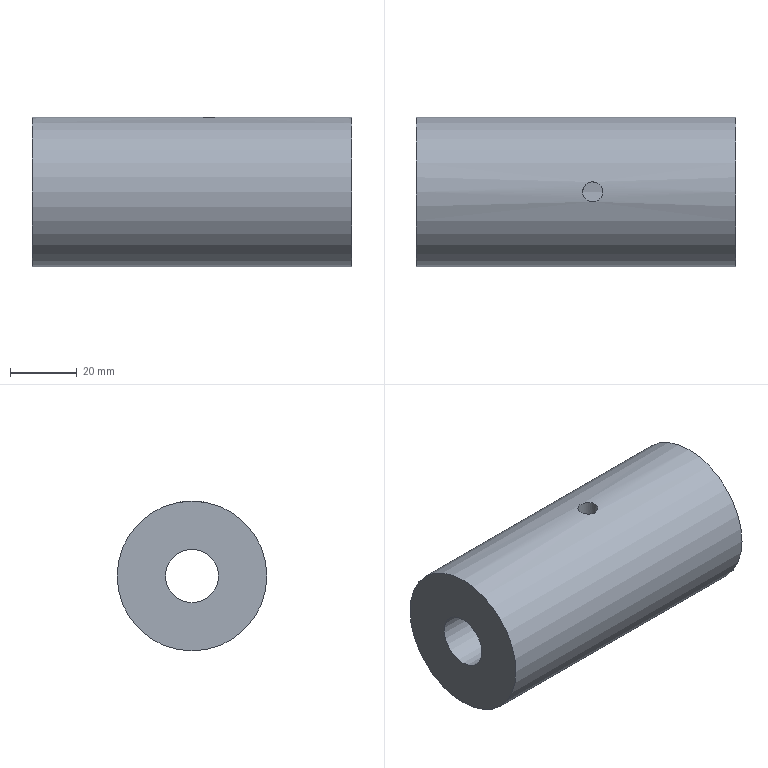Component | NX | FIXED_SLEEVE | 1 solid | 7 faces | volume 84940 mm3 | cylinder 4 | plane 3 | commonest cylinder face diameters 45 x1 32 x1 16 x1 6 x1